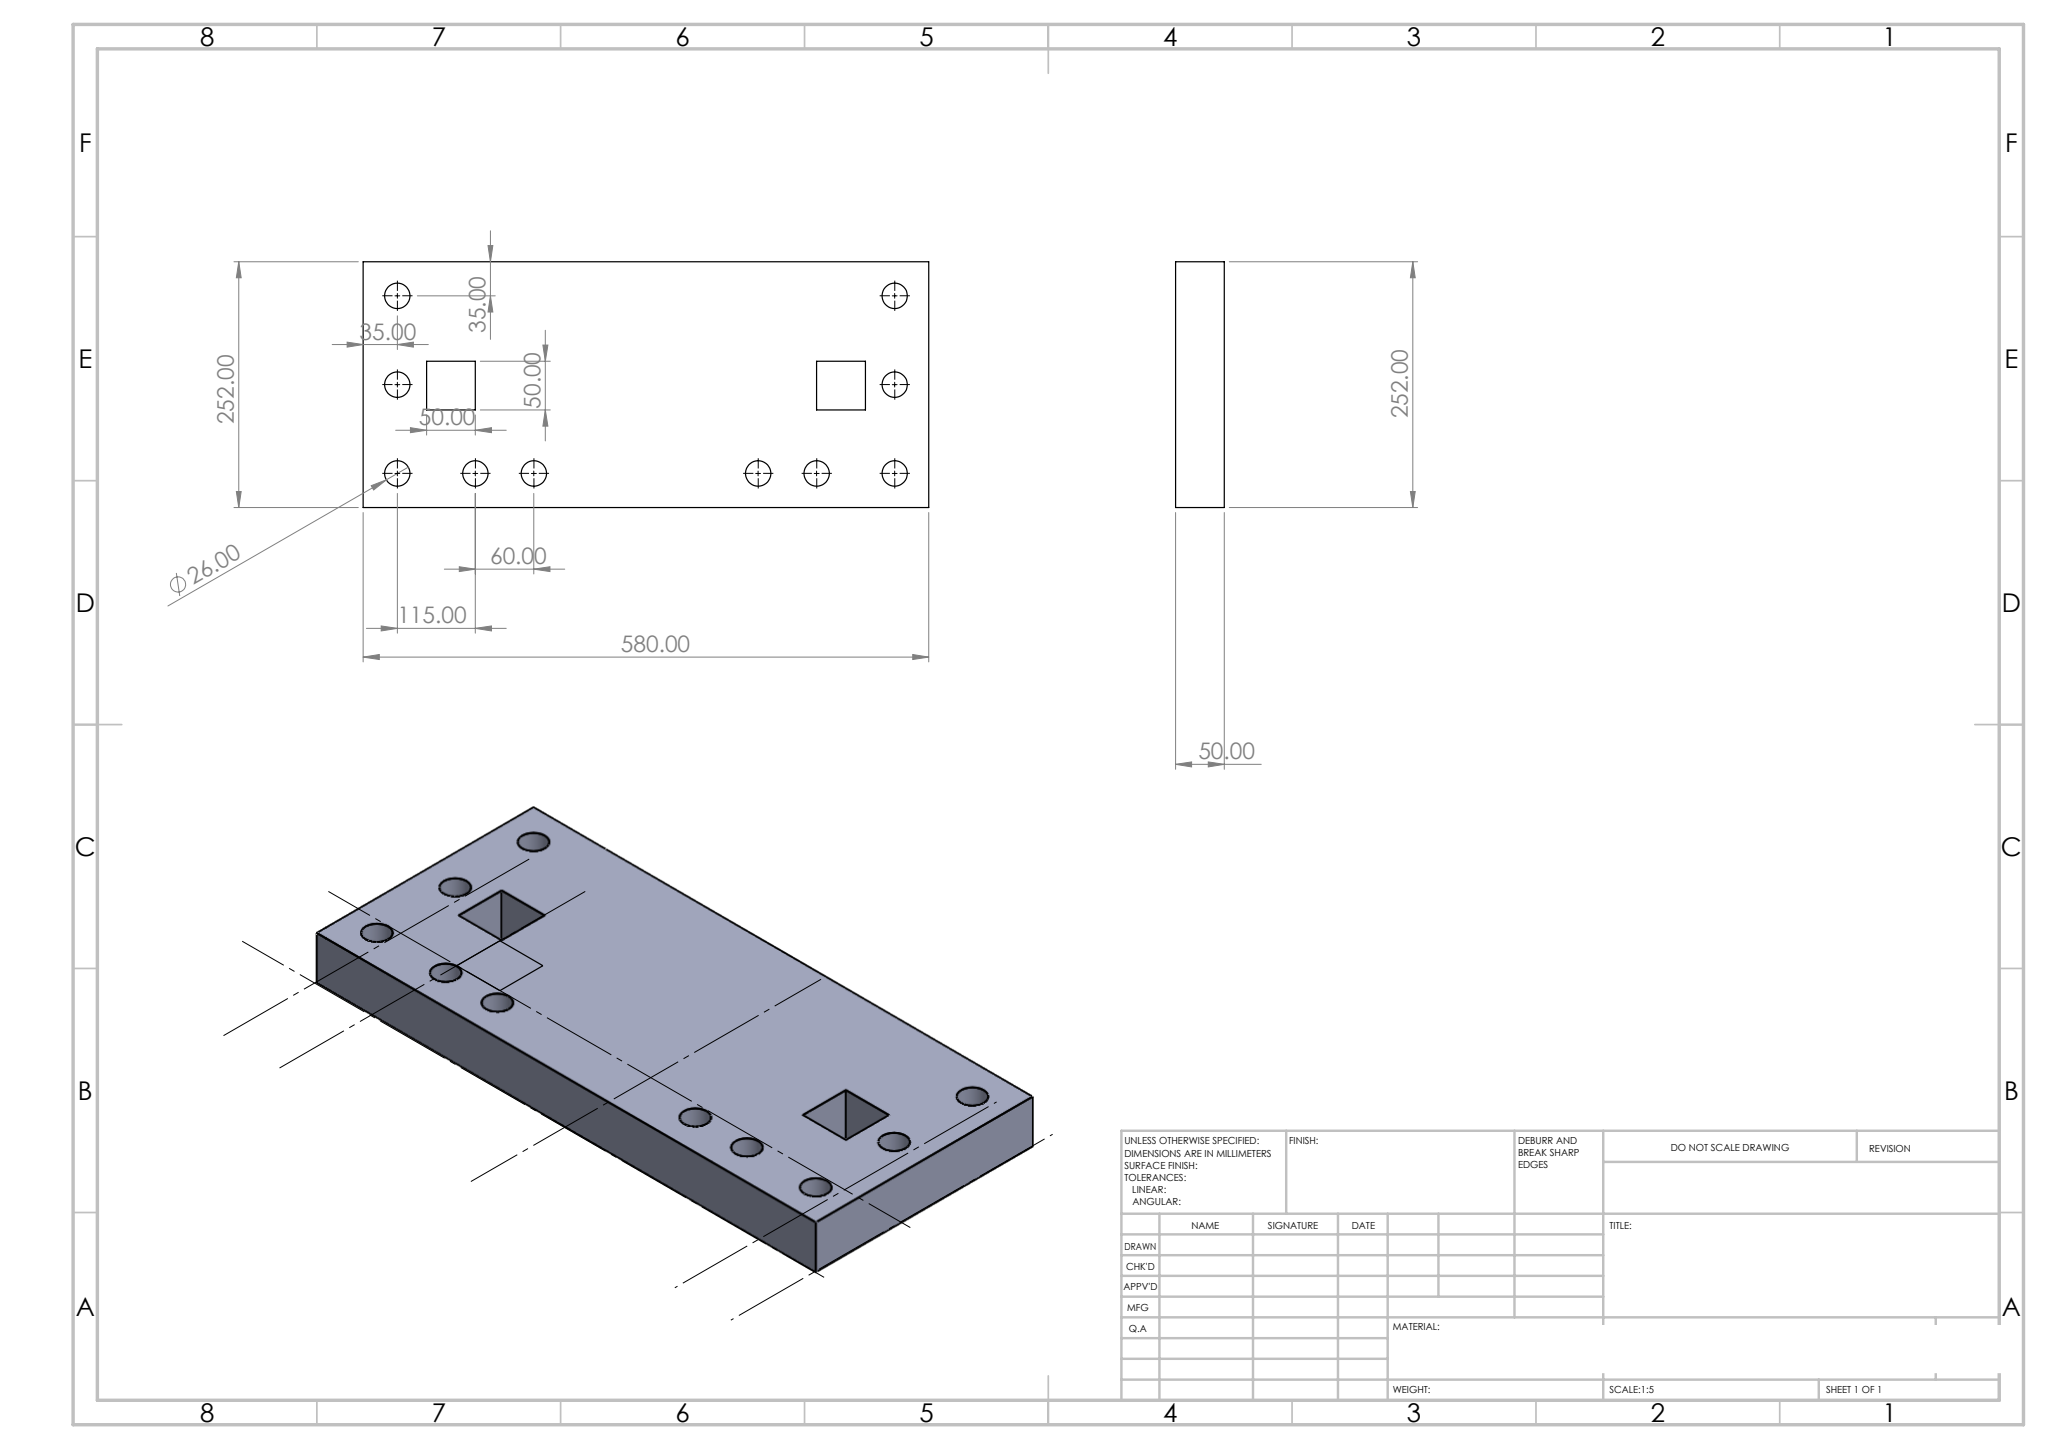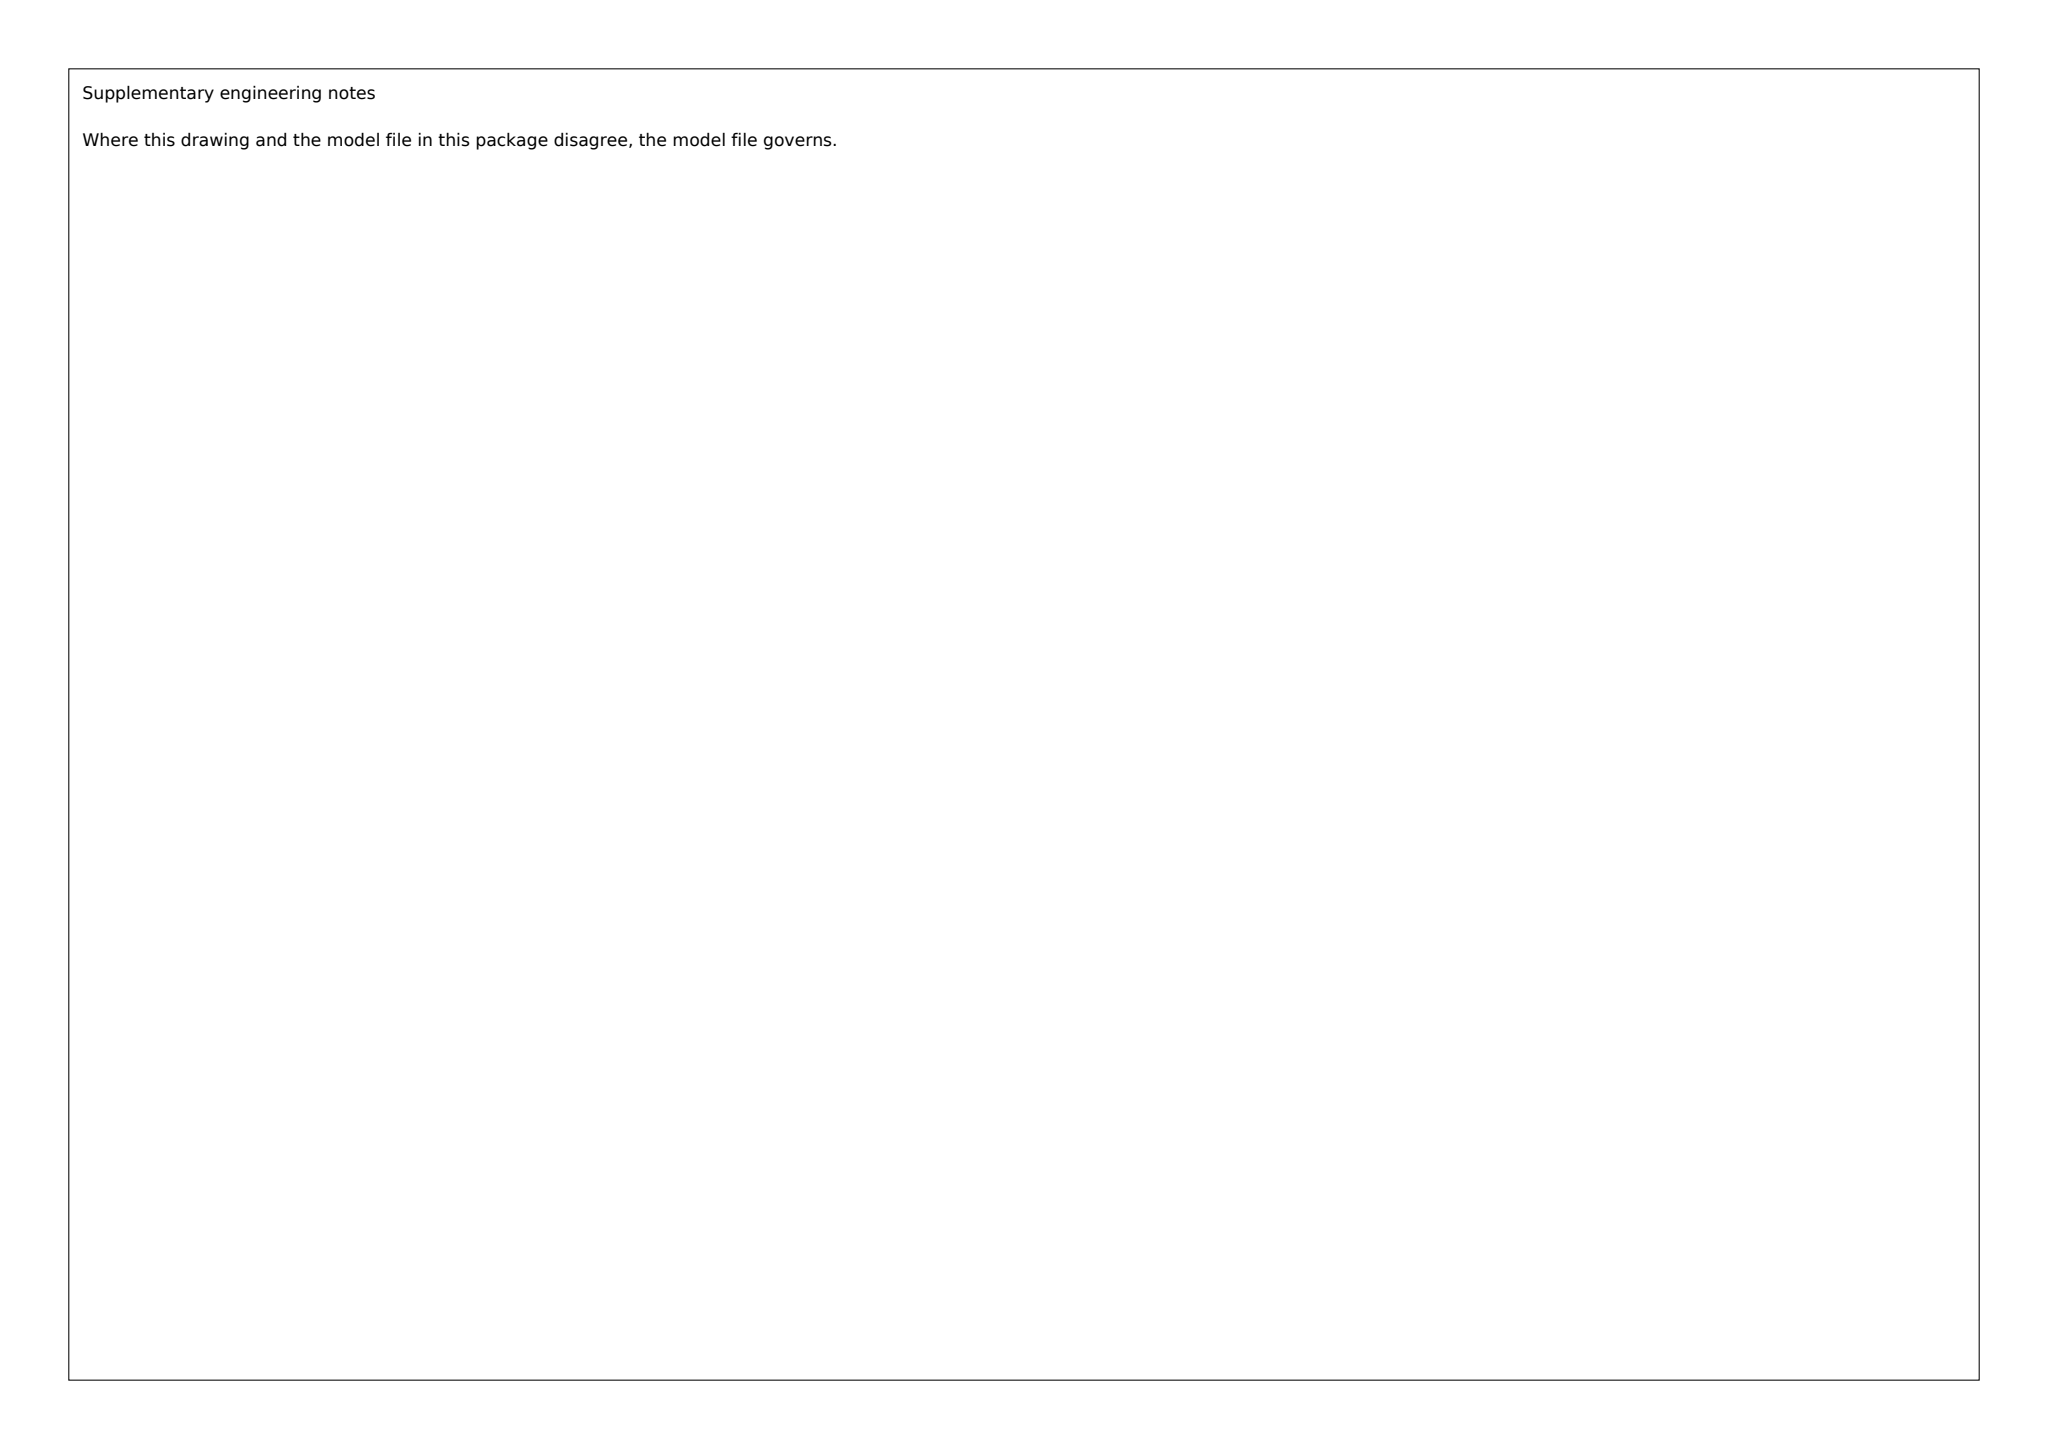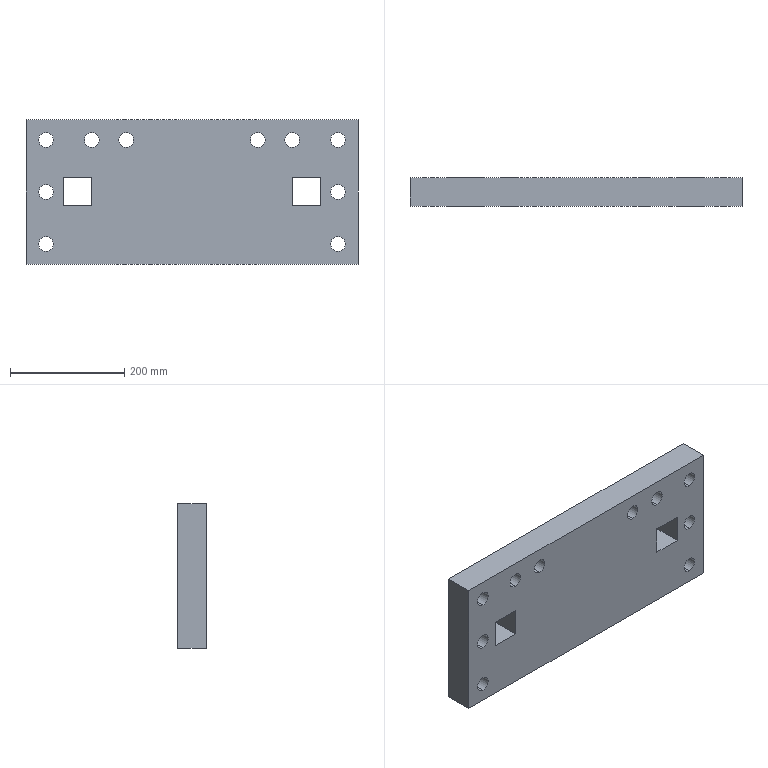Part | SolidWorks | mm | 1 solid | 34 faces | box 580 x 50 x 252 mm | volume 6792535 mm3 | cylinder 20 | plane 14 | commonest cylinder face diameters 26 x20
build123d program:
from build123d import *

# Parameters (mm, degrees)
SKETCH2_W           = 580
SKETCH2_H           = 252
SKETCH2_R           = 13
BOSS_EXTRUDE1_DEPTH = 50
SKETCH9_W           = 50
SKETCH9_H           = 50
CUT_EXTRUDE11_DEPTH = 321.119


with BuildPart() as part:
    # Sketch2 → Boss-Extrude1 (new body)
    with BuildSketch(Plane(origin=(0, 0, 0), x_dir=(1, 0, 0), z_dir=(0, 1, 0))):
        Rectangle(SKETCH2_W, SKETCH2_H)
        with Locations(Location((-255, -91, 0), (0, 0, 270))):
            Circle(SKETCH2_R, mode=Mode.SUBTRACT)
        with Locations(Location((-175, -91, 0), (0, 0, 270))):
            Circle(SKETCH2_R, mode=Mode.SUBTRACT)
        with Locations(Location((-115, -91, 0), (0, 0, 270))):
            Circle(SKETCH2_R, mode=Mode.SUBTRACT)
        with Locations(Location((-255, 0, 0), (0, 0, 270))):
            Circle(SKETCH2_R, mode=Mode.SUBTRACT)
        with Locations(Location((-255, 91, 0), (0, 0, 270))):
            Circle(SKETCH2_R, mode=Mode.SUBTRACT)
        with Locations(Location((115, -91, 0), (0, 0, 90))):
            Circle(SKETCH2_R, mode=Mode.SUBTRACT)
        with Locations(Location((175, -91, 0), (0, 0, 90))):
            Circle(SKETCH2_R, mode=Mode.SUBTRACT)
        with Locations(Location((255, -91, 0), (0, 0, 90))):
            Circle(SKETCH2_R, mode=Mode.SUBTRACT)
        with Locations(Location((255, 0, 0), (0, 0, 90))):
            Circle(SKETCH2_R, mode=Mode.SUBTRACT)
        with Locations(Location((255, 91, 0), (0, 0, 90))):
            Circle(SKETCH2_R, mode=Mode.SUBTRACT)
    extrude(amount=BOSS_EXTRUDE1_DEPTH)

    # Sketch9 → Cut-Extrude11 (cut, through all)
    with BuildSketch(Plane(origin=(0, 50, 0), x_dir=(1, 0, 0), z_dir=(0, 1, 0))):
        with Locations((-200, -1)):
            Rectangle(SKETCH9_W, SKETCH9_H)
        with Locations((200, -1)):
            Rectangle(SKETCH9_W, SKETCH9_H)
    extrude(amount=-CUT_EXTRUDE11_DEPTH, mode=Mode.SUBTRACT)


solid = part.part